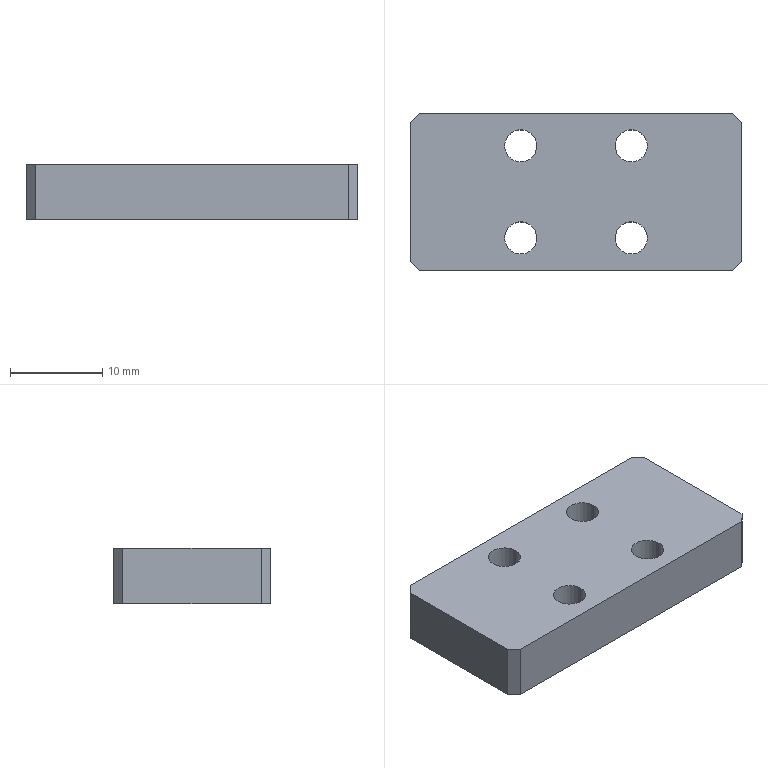Component | SolidWorks | ClampC-1 | 1 solid | 18 faces | box 36 x 17 x 6 mm | volume 3429 mm3 | plane 10 | cylinder 8 | commonest cylinder face diameters 3.5 x8
build123d program:
from build123d import *

# Parameters (mm, degrees)
SKETCH1_W                  = 36
SKETCH1_H                  = 17
EXTRUDE1_DEPTH             = 6
F_3_5_3_5_DIAMETER_HOLE1_D = 3.5
CHAMFER1_SIZE              = 1


with BuildPart() as part:
    # Sketch1 → Extrude1 (new body)
    with BuildSketch(Plane.XY):
        Rectangle(SKETCH1_W, SKETCH1_H)
    extrude(amount=EXTRUDE1_DEPTH)

    # 3.5 _3.5_ Diameter Hole1 (through all)
    with Locations(Plane.XY.offset(6)):
        with Locations((-6, 5), (6, 5), (6, -5), (-6, -5)):
            Hole(F_3_5_3_5_DIAMETER_HOLE1_D / 2)

    # Chamfer1
    chamfer1_edges = [part.edges().sort_by_distance(p)[0] for p in [
        (-18, 8.5, 3),
        (18, 8.5, 3),
        (18, -8.5, 3),
        (-18, -8.5, 3),
    ]]
    chamfer(chamfer1_edges, length=CHAMFER1_SIZE)


solid = part.part

# Placed as in the assembly
solid = solid.moved(Location((13, 29, 10), (0, 0, 0)))
STEP:
#1=CARTESIAN_POINT('',(0.2067,1.339,0.3937));
#2=VERTEX_POINT('',#1);
#3=CARTESIAN_POINT('',(0.3445,1.339,0.3937));
#4=VERTEX_POINT('',#3);
#5=CARTESIAN_POINT('',(0.2756,1.339,0.3937));
#6=DIRECTION('',(0.,0.,1.));
#7=DIRECTION('',(1.,0.,0.));
#8=AXIS2_PLACEMENT_3D('',#5,#6,#7);
#9=CIRCLE('',#8,0.0689);
#10=EDGE_CURVE('',#2,#4,#9,.T.);
#11=ORIENTED_EDGE('',*,*,#10,.F.);
#12=CARTESIAN_POINT('',(0.2067,1.339,0.6299));
#13=VERTEX_POINT('',#12);
#14=CARTESIAN_POINT('',(0.2067,1.339,0.6299));
#15=DIRECTION('',(0.,0.,1.));
#16=VECTOR('',#15,39.37);
#17=LINE('',#14,#16);
#18=EDGE_CURVE('',#2,#13,#17,.T.);
#19=ORIENTED_EDGE('',*,*,#18,.T.);
#20=CARTESIAN_POINT('',(0.3445,1.339,0.6299));
#21=VERTEX_POINT('',#20);
#22=CARTESIAN_POINT('',(0.2756,1.339,0.6299));
#23=DIRECTION('',(0.,0.,1.));
#24=DIRECTION('',(1.,0.,0.));
#25=AXIS2_PLACEMENT_3D('',#22,#23,#24);
#26=CIRCLE('',#25,0.0689);
#27=EDGE_CURVE('',#13,#21,#26,.T.);
#28=ORIENTED_EDGE('',*,*,#27,.T.);
#29=CARTESIAN_POINT('',(0.3445,1.339,0.6299));
#30=DIRECTION('',(0.,0.,1.));
#31=VECTOR('',#30,39.37);
#32=LINE('',#29,#31);
#33=EDGE_CURVE('',#4,#21,#32,.T.);
#34=ORIENTED_EDGE('',*,*,#33,.F.);
#35=EDGE_LOOP('',(#11,#19,#28,#34));
#36=FACE_OUTER_BOUND('',#35,.T.);
#37=CARTESIAN_POINT('',(0.2756,1.339,0.6299));
#38=DIRECTION('',(0.,0.,1.));
#39=DIRECTION('',(1.,0.,0.));
#40=AXIS2_PLACEMENT_3D('',#37,#38,#39);
#41=CYLINDRICAL_SURFACE('',#40,0.0689);
#42=ADVANCED_FACE('',(#36),#41,.F.);
#43=CARTESIAN_POINT('',(0.6791,1.339,0.3937));
#44=VERTEX_POINT('',#43);
#45=CARTESIAN_POINT('',(0.8169,1.339,0.3937));
#46=VERTEX_POINT('',#45);
#47=CARTESIAN_POINT('',(0.748,1.339,0.3937));
#48=DIRECTION('',(0.,0.,1.));
#49=DIRECTION('',(1.,0.,0.));
#50=AXIS2_PLACEMENT_3D('',#47,#48,#49);
#51=CIRCLE('',#50,0.0689);
#52=EDGE_CURVE('',#44,#46,#51,.T.);
#53=ORIENTED_EDGE('',*,*,#52,.F.);
#54=CARTESIAN_POINT('',(0.6791,1.339,0.6299));
#55=VERTEX_POINT('',#54);
#56=CARTESIAN_POINT('',(0.6791,1.339,0.6299));
#57=DIRECTION('',(0.,0.,1.));
#58=VECTOR('',#57,39.37);
#59=LINE('',#56,#58);
#60=EDGE_CURVE('',#44,#55,#59,.T.);
#61=ORIENTED_EDGE('',*,*,#60,.T.);
#62=CARTESIAN_POINT('',(0.8169,1.339,0.6299));
#63=VERTEX_POINT('',#62);
#64=CARTESIAN_POINT('',(0.748,1.339,0.6299));
#65=DIRECTION('',(0.,0.,1.));
#66=DIRECTION('',(1.,0.,0.));
#67=AXIS2_PLACEMENT_3D('',#64,#65,#66);
#68=CIRCLE('',#67,0.0689);
#69=EDGE_CURVE('',#55,#63,#68,.T.);
#70=ORIENTED_EDGE('',*,*,#69,.T.);
#71=CARTESIAN_POINT('',(0.8169,1.339,0.6299));
#72=DIRECTION('',(0.,0.,1.));
#73=VECTOR('',#72,39.37);
#74=LINE('',#71,#73);
#75=EDGE_CURVE('',#46,#63,#74,.T.);
#76=ORIENTED_EDGE('',*,*,#75,.F.);
#77=EDGE_LOOP('',(#53,#61,#70,#76));
#78=FACE_OUTER_BOUND('',#77,.T.);
#79=CARTESIAN_POINT('',(0.748,1.339,0.6299));
#80=DIRECTION('',(0.,0.,1.));
#81=DIRECTION('',(1.,0.,0.));
#82=AXIS2_PLACEMENT_3D('',#79,#80,#81);
#83=CYLINDRICAL_SURFACE('',#82,0.0689);
#84=ADVANCED_FACE('',(#78),#83,.F.);
#85=CARTESIAN_POINT('',(0.6791,0.9449,0.3937));
#86=VERTEX_POINT('',#85);
#87=CARTESIAN_POINT('',(0.8169,0.9449,0.3937));
#88=VERTEX_POINT('',#87);
#89=CARTESIAN_POINT('',(0.748,0.9449,0.3937));
#90=DIRECTION('',(0.,0.,1.));
#91=DIRECTION('',(1.,0.,0.));
#92=AXIS2_PLACEMENT_3D('',#89,#90,#91);
#93=CIRCLE('',#92,0.0689);
#94=EDGE_CURVE('',#86,#88,#93,.T.);
#95=ORIENTED_EDGE('',*,*,#94,.F.);
#96=CARTESIAN_POINT('',(0.6791,0.9449,0.6299));
#97=VERTEX_POINT('',#96);
#98=CARTESIAN_POINT('',(0.6791,0.9449,0.6299));
#99=DIRECTION('',(0.,0.,1.));
#100=VECTOR('',#99,39.37);
#101=LINE('',#98,#100);
#102=EDGE_CURVE('',#86,#97,#101,.T.);
#103=ORIENTED_EDGE('',*,*,#102,.T.);
#104=CARTESIAN_POINT('',(0.8169,0.9449,0.6299));
#105=VERTEX_POINT('',#104);
#106=CARTESIAN_POINT('',(0.748,0.9449,0.6299));
#107=DIRECTION('',(0.,0.,1.));
#108=DIRECTION('',(1.,0.,0.));
#109=AXIS2_PLACEMENT_3D('',#106,#107,#108);
#110=CIRCLE('',#109,0.0689);
#111=EDGE_CURVE('',#97,#105,#110,.T.);
#112=ORIENTED_EDGE('',*,*,#111,.T.);
#113=CARTESIAN_POINT('',(0.8169,0.9449,0.6299));
#114=DIRECTION('',(0.,0.,1.));
#115=VECTOR('',#114,39.37);
#116=LINE('',#113,#115);
#117=EDGE_CURVE('',#88,#105,#116,.T.);
#118=ORIENTED_EDGE('',*,*,#117,.F.);
#119=EDGE_LOOP('',(#95,#103,#112,#118));
#120=FACE_OUTER_BOUND('',#119,.T.);
#121=CARTESIAN_POINT('',(0.748,0.9449,0.6299));
#122=DIRECTION('',(0.,0.,1.));
#123=DIRECTION('',(1.,0.,0.));
#124=AXIS2_PLACEMENT_3D('',#121,#122,#123);
#125=CYLINDRICAL_SURFACE('',#124,0.0689);
#126=ADVANCED_FACE('',(#120),#125,.F.);
#127=CARTESIAN_POINT('',(0.2067,0.9449,0.3937));
#128=VERTEX_POINT('',#127);
#129=CARTESIAN_POINT('',(0.3445,0.9449,0.3937));
#130=VERTEX_POINT('',#129);
#131=CARTESIAN_POINT('',(0.2756,0.9449,0.3937));
#132=DIRECTION('',(0.,0.,1.));
#133=DIRECTION('',(1.,0.,0.));
#134=AXIS2_PLACEMENT_3D('',#131,#132,#133);
#135=CIRCLE('',#134,0.0689);
#136=EDGE_CURVE('',#128,#130,#135,.T.);
#137=ORIENTED_EDGE('',*,*,#136,.F.);
#138=CARTESIAN_POINT('',(0.2067,0.9449,0.6299));
#139=VERTEX_POINT('',#138);
#140=CARTESIAN_POINT('',(0.2067,0.9449,0.6299));
#141=DIRECTION('',(0.,0.,1.));
#142=VECTOR('',#141,39.37);
#143=LINE('',#140,#142);
#144=EDGE_CURVE('',#128,#139,#143,.T.);
#145=ORIENTED_EDGE('',*,*,#144,.T.);
#146=CARTESIAN_POINT('',(0.3445,0.9449,0.6299));
#147=VERTEX_POINT('',#146);
#148=CARTESIAN_POINT('',(0.2756,0.9449,0.6299));
#149=DIRECTION('',(0.,0.,1.));
#150=DIRECTION('',(1.,0.,0.));
#151=AXIS2_PLACEMENT_3D('',#148,#149,#150);
#152=CIRCLE('',#151,0.0689);
#153=EDGE_CURVE('',#139,#147,#152,.T.);
#154=ORIENTED_EDGE('',*,*,#153,.T.);
#155=CARTESIAN_POINT('',(0.3445,0.9449,0.6299));
#156=DIRECTION('',(0.,0.,1.));
#157=VECTOR('',#156,39.37);
#158=LINE('',#155,#157);
#159=EDGE_CURVE('',#130,#147,#158,.T.);
#160=ORIENTED_EDGE('',*,*,#159,.F.);
#161=EDGE_LOOP('',(#137,#145,#154,#160));
#162=FACE_OUTER_BOUND('',#161,.T.);
#163=CARTESIAN_POINT('',(0.2756,0.9449,0.6299));
#164=DIRECTION('',(0.,0.,1.));
#165=DIRECTION('',(1.,0.,0.));
#166=AXIS2_PLACEMENT_3D('',#163,#164,#165);
#167=CYLINDRICAL_SURFACE('',#166,0.0689);
#168=ADVANCED_FACE('',(#162),#167,.F.);
#169=CARTESIAN_POINT('',(-0.1969,1.437,0.3937));
#170=VERTEX_POINT('',#169);
#171=CARTESIAN_POINT('',(-0.1969,0.8465,0.3937));
#172=VERTEX_POINT('',#171);
#173=CARTESIAN_POINT('',(-0.1969,0.8071,0.3937));
#174=DIRECTION('',(0.,-1.,0.));
#175=VECTOR('',#174,39.37);
#176=LINE('',#173,#175);
#177=EDGE_CURVE('',#170,#172,#176,.T.);
#178=ORIENTED_EDGE('',*,*,#177,.T.);
#179=CARTESIAN_POINT('',(-0.1969,0.8465,0.6299));
#180=VERTEX_POINT('',#179);
#181=CARTESIAN_POINT('',(-0.1969,0.8465,0.6299));
#182=DIRECTION('',(0.,0.,1.));
#183=VECTOR('',#182,39.37);
#184=LINE('',#181,#183);
#185=EDGE_CURVE('',#172,#180,#184,.T.);
#186=ORIENTED_EDGE('',*,*,#185,.T.);
#187=CARTESIAN_POINT('',(-0.1969,1.437,0.6299));
#188=VERTEX_POINT('',#187);
#189=CARTESIAN_POINT('',(-0.1969,0.8071,0.6299));
#190=DIRECTION('',(0.,-1.,0.));
#191=VECTOR('',#190,39.37);
#192=LINE('',#189,#191);
#193=EDGE_CURVE('',#188,#180,#192,.T.);
#194=ORIENTED_EDGE('',*,*,#193,.F.);
#195=CARTESIAN_POINT('',(-0.1969,1.437,0.6299));
#196=DIRECTION('',(0.,0.,-1.));
#197=VECTOR('',#196,39.37);
#198=LINE('',#195,#197);
#199=EDGE_CURVE('',#188,#170,#198,.T.);
#200=ORIENTED_EDGE('',*,*,#199,.T.);
#201=EDGE_LOOP('',(#178,#186,#194,#200));
#202=FACE_OUTER_BOUND('',#201,.T.);
#203=CARTESIAN_POINT('',(-0.1969,0.8071,0.6299));
#204=DIRECTION('',(1.,0.,0.));
#205=DIRECTION('',(0.,0.,-1.));
#206=AXIS2_PLACEMENT_3D('',#203,#204,#205);
#207=PLANE('',#206);
#208=ADVANCED_FACE('',(#202),#207,.F.);
#209=CARTESIAN_POINT('',(-0.1575,0.8071,0.3937));
#210=VERTEX_POINT('',#209);
#211=CARTESIAN_POINT('',(1.181,0.8071,0.3937));
#212=VERTEX_POINT('',#211);
#213=CARTESIAN_POINT('',(1.22,0.8071,0.3937));
#214=DIRECTION('',(1.,0.,0.));
#215=VECTOR('',#214,39.37);
#216=LINE('',#213,#215);
#217=EDGE_CURVE('',#210,#212,#216,.T.);
#218=ORIENTED_EDGE('',*,*,#217,.T.);
#219=CARTESIAN_POINT('',(1.181,0.8071,0.6299));
#220=VERTEX_POINT('',#219);
#221=CARTESIAN_POINT('',(1.181,0.8071,0.6299));
#222=DIRECTION('',(0.,0.,1.));
#223=VECTOR('',#222,39.37);
#224=LINE('',#221,#223);
#225=EDGE_CURVE('',#212,#220,#224,.T.);
#226=ORIENTED_EDGE('',*,*,#225,.T.);
#227=CARTESIAN_POINT('',(-0.1575,0.8071,0.6299));
#228=VERTEX_POINT('',#227);
#229=CARTESIAN_POINT('',(1.22,0.8071,0.6299));
#230=DIRECTION('',(1.,0.,0.));
#231=VECTOR('',#230,39.37);
#232=LINE('',#229,#231);
#233=EDGE_CURVE('',#228,#220,#232,.T.);
#234=ORIENTED_EDGE('',*,*,#233,.F.);
#235=CARTESIAN_POINT('',(-0.1575,0.8071,0.6299));
#236=DIRECTION('',(0.,0.,-1.));
#237=VECTOR('',#236,39.37);
#238=LINE('',#235,#237);
#239=EDGE_CURVE('',#228,#210,#238,.T.);
#240=ORIENTED_EDGE('',*,*,#239,.T.);
#241=EDGE_LOOP('',(#218,#226,#234,#240));
#242=FACE_OUTER_BOUND('',#241,.T.);
#243=CARTESIAN_POINT('',(1.22,0.8071,0.6299));
#244=DIRECTION('',(-0.,1.,0.));
#245=DIRECTION('',(-1.,-0.,0.));
#246=AXIS2_PLACEMENT_3D('',#243,#244,#245);
#247=PLANE('',#246);
#248=ADVANCED_FACE('',(#242),#247,.F.);
#249=CARTESIAN_POINT('',(1.22,0.8465,0.6299));
#250=VERTEX_POINT('',#249);
#251=CARTESIAN_POINT('',(1.22,1.437,0.6299));
#252=VERTEX_POINT('',#251);
#253=CARTESIAN_POINT('',(1.22,0.8071,0.6299));
#254=DIRECTION('',(0.,1.,0.));
#255=VECTOR('',#254,39.37);
#256=LINE('',#253,#255);
#257=EDGE_CURVE('',#250,#252,#256,.T.);
#258=ORIENTED_EDGE('',*,*,#257,.F.);
#259=CARTESIAN_POINT('',(1.22,0.8465,0.3937));
#260=VERTEX_POINT('',#259);
#261=CARTESIAN_POINT('',(1.22,0.8465,0.6299));
#262=DIRECTION('',(0.,0.,-1.));
#263=VECTOR('',#262,39.37);
#264=LINE('',#261,#263);
#265=EDGE_CURVE('',#250,#260,#264,.T.);
#266=ORIENTED_EDGE('',*,*,#265,.T.);
#267=CARTESIAN_POINT('',(1.22,1.437,0.3937));
#268=VERTEX_POINT('',#267);
#269=CARTESIAN_POINT('',(1.22,0.8071,0.3937));
#270=DIRECTION('',(0.,1.,0.));
#271=VECTOR('',#270,39.37);
#272=LINE('',#269,#271);
#273=EDGE_CURVE('',#260,#268,#272,.T.);
#274=ORIENTED_EDGE('',*,*,#273,.T.);
#275=CARTESIAN_POINT('',(1.22,1.437,0.6299));
#276=DIRECTION('',(0.,0.,1.));
#277=VECTOR('',#276,39.37);
#278=LINE('',#275,#277);
#279=EDGE_CURVE('',#268,#252,#278,.T.);
#280=ORIENTED_EDGE('',*,*,#279,.T.);
#281=EDGE_LOOP('',(#258,#266,#274,#280));
#282=FACE_OUTER_BOUND('',#281,.T.);
#283=CARTESIAN_POINT('',(1.22,0.8071,0.6299));
#284=DIRECTION('',(-1.,0.,0.));
#285=DIRECTION('',(0.,0.,1.));
#286=AXIS2_PLACEMENT_3D('',#283,#284,#285);
#287=PLANE('',#286);
#288=ADVANCED_FACE('',(#282),#287,.F.);
#289=CARTESIAN_POINT('',(1.181,1.476,0.6299));
#290=VERTEX_POINT('',#289);
#291=CARTESIAN_POINT('',(-0.1575,1.476,0.6299));
#292=VERTEX_POINT('',#291);
#293=CARTESIAN_POINT('',(1.22,1.476,0.6299));
#294=DIRECTION('',(-1.,-0.,0.));
#295=VECTOR('',#294,39.37);
#296=LINE('',#293,#295);
#297=EDGE_CURVE('',#290,#292,#296,.T.);
#298=ORIENTED_EDGE('',*,*,#297,.F.);
#299=CARTESIAN_POINT('',(1.181,1.476,0.3937));
#300=VERTEX_POINT('',#299);
#301=CARTESIAN_POINT('',(1.181,1.476,0.6299));
#302=DIRECTION('',(0.,0.,-1.));
#303=VECTOR('',#302,39.37);
#304=LINE('',#301,#303);
#305=EDGE_CURVE('',#290,#300,#304,.T.);
#306=ORIENTED_EDGE('',*,*,#305,.T.);
#307=CARTESIAN_POINT('',(-0.1575,1.476,0.3937));
#308=VERTEX_POINT('',#307);
#309=CARTESIAN_POINT('',(1.22,1.476,0.3937));
#310=DIRECTION('',(-1.,-0.,0.));
#311=VECTOR('',#310,39.37);
#312=LINE('',#309,#311);
#313=EDGE_CURVE('',#300,#308,#312,.T.);
#314=ORIENTED_EDGE('',*,*,#313,.T.);
#315=CARTESIAN_POINT('',(-0.1575,1.476,0.6299));
#316=DIRECTION('',(0.,0.,1.));
#317=VECTOR('',#316,39.37);
#318=LINE('',#315,#317);
#319=EDGE_CURVE('',#308,#292,#318,.T.);
#320=ORIENTED_EDGE('',*,*,#319,.T.);
#321=EDGE_LOOP('',(#298,#306,#314,#320));
#322=FACE_OUTER_BOUND('',#321,.T.);
#323=CARTESIAN_POINT('',(1.22,1.476,0.6299));
#324=DIRECTION('',(0.,-1.,0.));
#325=DIRECTION('',(1.,0.,0.));
#326=AXIS2_PLACEMENT_3D('',#323,#324,#325);
#327=PLANE('',#326);
#328=ADVANCED_FACE('',(#322),#327,.F.);
#329=CARTESIAN_POINT('',(0.2756,1.339,0.6299));
#330=DIRECTION('',(0.,0.,1.));
#331=DIRECTION('',(1.,0.,0.));
#332=AXIS2_PLACEMENT_3D('',#329,#330,#331);
#333=CIRCLE('',#332,0.0689);
#334=EDGE_CURVE('',#21,#13,#333,.T.);
#335=ORIENTED_EDGE('',*,*,#334,.F.);
#336=ORIENTED_EDGE('',*,*,#27,.F.);
#337=EDGE_LOOP('',(#335,#336));
#338=FACE_BOUND('',#337,.T.);
#339=CARTESIAN_POINT('',(0.748,1.339,0.6299));
#340=DIRECTION('',(0.,0.,1.));
#341=DIRECTION('',(1.,0.,0.));
#342=AXIS2_PLACEMENT_3D('',#339,#340,#341);
#343=CIRCLE('',#342,0.0689);
#344=EDGE_CURVE('',#63,#55,#343,.T.);
#345=ORIENTED_EDGE('',*,*,#344,.F.);
#346=ORIENTED_EDGE('',*,*,#69,.F.);
#347=EDGE_LOOP('',(#345,#346));
#348=FACE_BOUND('',#347,.T.);
#349=CARTESIAN_POINT('',(0.748,0.9449,0.6299));
#350=DIRECTION('',(0.,0.,1.));
#351=DIRECTION('',(1.,0.,0.));
#352=AXIS2_PLACEMENT_3D('',#349,#350,#351);
#353=CIRCLE('',#352,0.0689);
#354=EDGE_CURVE('',#105,#97,#353,.T.);
#355=ORIENTED_EDGE('',*,*,#354,.F.);
#356=ORIENTED_EDGE('',*,*,#111,.F.);
#357=EDGE_LOOP('',(#355,#356));
#358=FACE_BOUND('',#357,.T.);
#359=CARTESIAN_POINT('',(0.2756,0.9449,0.6299));
#360=DIRECTION('',(0.,0.,1.));
#361=DIRECTION('',(1.,0.,0.));
#362=AXIS2_PLACEMENT_3D('',#359,#360,#361);
#363=CIRCLE('',#362,0.0689);
#364=EDGE_CURVE('',#147,#139,#363,.T.);
#365=ORIENTED_EDGE('',*,*,#364,.F.);
#366=ORIENTED_EDGE('',*,*,#153,.F.);
#367=EDGE_LOOP('',(#365,#366));
#368=FACE_BOUND('',#367,.T.);
#369=ORIENTED_EDGE('',*,*,#233,.T.);
#370=CARTESIAN_POINT('',(0.8268,0.4528,0.6299));
#371=DIRECTION('',(0.7071,0.7071,0.));
#372=VECTOR('',#371,39.37);
#373=LINE('',#370,#372);
#374=EDGE_CURVE('',#220,#250,#373,.T.);
#375=ORIENTED_EDGE('',*,*,#374,.T.);
#376=ORIENTED_EDGE('',*,*,#257,.T.);
#377=CARTESIAN_POINT('',(0.4921,2.165,0.6299));
#378=DIRECTION('',(-0.7071,0.7071,0.));
#379=VECTOR('',#378,39.37);
#380=LINE('',#377,#379);
#381=EDGE_CURVE('',#252,#290,#380,.T.);
#382=ORIENTED_EDGE('',*,*,#381,.T.);
#383=ORIENTED_EDGE('',*,*,#297,.T.);
#384=CARTESIAN_POINT('',(-0.1772,1.457,0.6299));
#385=DIRECTION('',(-0.7071,-0.7071,0.));
#386=VECTOR('',#385,39.37);
#387=LINE('',#384,#386);
#388=EDGE_CURVE('',#292,#188,#387,.T.);
#389=ORIENTED_EDGE('',*,*,#388,.T.);
#390=ORIENTED_EDGE('',*,*,#193,.T.);
#391=CARTESIAN_POINT('',(-0.5118,1.161,0.6299));
#392=DIRECTION('',(0.7071,-0.7071,0.));
#393=VECTOR('',#392,39.37);
#394=LINE('',#391,#393);
#395=EDGE_CURVE('',#180,#228,#394,.T.);
#396=ORIENTED_EDGE('',*,*,#395,.T.);
#397=EDGE_LOOP('',(#369,#375,#376,#382,#383,#389,#390,#396));
#398=FACE_OUTER_BOUND('',#397,.T.);
#399=CARTESIAN_POINT('',(-0.1969,1.476,0.6299));
#400=DIRECTION('',(0.,0.,1.));
#401=DIRECTION('',(1.,0.,0.));
#402=AXIS2_PLACEMENT_3D('',#399,#400,#401);
#403=PLANE('',#402);
#404=ADVANCED_FACE('',(#338,#348,#358,#368,#398),#403,.T.);
#405=CARTESIAN_POINT('',(0.2756,1.339,0.3937));
#406=DIRECTION('',(0.,0.,1.));
#407=DIRECTION('',(1.,0.,0.));
#408=AXIS2_PLACEMENT_3D('',#405,#406,#407);
#409=CIRCLE('',#408,0.0689);
#410=EDGE_CURVE('',#4,#2,#409,.T.);
#411=ORIENTED_EDGE('',*,*,#410,.T.);
#412=ORIENTED_EDGE('',*,*,#10,.T.);
#413=EDGE_LOOP('',(#411,#412));
#414=FACE_BOUND('',#413,.T.);
#415=CARTESIAN_POINT('',(0.748,1.339,0.3937));
#416=DIRECTION('',(0.,0.,1.));
#417=DIRECTION('',(1.,0.,0.));
#418=AXIS2_PLACEMENT_3D('',#415,#416,#417);
#419=CIRCLE('',#418,0.0689);
#420=EDGE_CURVE('',#46,#44,#419,.T.);
#421=ORIENTED_EDGE('',*,*,#420,.T.);
#422=ORIENTED_EDGE('',*,*,#52,.T.);
#423=EDGE_LOOP('',(#421,#422));
#424=FACE_BOUND('',#423,.T.);
#425=CARTESIAN_POINT('',(0.748,0.9449,0.3937));
#426=DIRECTION('',(0.,0.,1.));
#427=DIRECTION('',(1.,0.,0.));
#428=AXIS2_PLACEMENT_3D('',#425,#426,#427);
#429=CIRCLE('',#428,0.0689);
#430=EDGE_CURVE('',#88,#86,#429,.T.);
#431=ORIENTED_EDGE('',*,*,#430,.T.);
#432=ORIENTED_EDGE('',*,*,#94,.T.);
#433=EDGE_LOOP('',(#431,#432));
#434=FACE_BOUND('',#433,.T.);
#435=CARTESIAN_POINT('',(0.2756,0.9449,0.3937));
#436=DIRECTION('',(0.,0.,1.));
#437=DIRECTION('',(1.,0.,0.));
#438=AXIS2_PLACEMENT_3D('',#435,#436,#437);
#439=CIRCLE('',#438,0.0689);
#440=EDGE_CURVE('',#130,#128,#439,.T.);
#441=ORIENTED_EDGE('',*,*,#440,.T.);
#442=ORIENTED_EDGE('',*,*,#136,.T.);
#443=EDGE_LOOP('',(#441,#442));
#444=FACE_BOUND('',#443,.T.);
#445=ORIENTED_EDGE('',*,*,#273,.F.);
#446=CARTESIAN_POINT('',(1.22,0.8465,0.3937));
#447=DIRECTION('',(-0.7071,-0.7071,0.));
#448=VECTOR('',#447,39.37);
#449=LINE('',#446,#448);
#450=EDGE_CURVE('',#260,#212,#449,.T.);
#451=ORIENTED_EDGE('',*,*,#450,.T.);
#452=ORIENTED_EDGE('',*,*,#217,.F.);
#453=CARTESIAN_POINT('',(-0.1575,0.8071,0.3937));
#454=DIRECTION('',(-0.7071,0.7071,0.));
#455=VECTOR('',#454,39.37);
#456=LINE('',#453,#455);
#457=EDGE_CURVE('',#210,#172,#456,.T.);
#458=ORIENTED_EDGE('',*,*,#457,.T.);
#459=ORIENTED_EDGE('',*,*,#177,.F.);
#460=CARTESIAN_POINT('',(-0.1969,1.437,0.3937));
#461=DIRECTION('',(0.7071,0.7071,0.));
#462=VECTOR('',#461,39.37);
#463=LINE('',#460,#462);
#464=EDGE_CURVE('',#170,#308,#463,.T.);
#465=ORIENTED_EDGE('',*,*,#464,.T.);
#466=ORIENTED_EDGE('',*,*,#313,.F.);
#467=CARTESIAN_POINT('',(1.181,1.476,0.3937));
#468=DIRECTION('',(0.7071,-0.7071,0.));
#469=VECTOR('',#468,39.37);
#470=LINE('',#467,#469);
#471=EDGE_CURVE('',#300,#268,#470,.T.);
#472=ORIENTED_EDGE('',*,*,#471,.T.);
#473=EDGE_LOOP('',(#445,#451,#452,#458,#459,#465,#466,#472));
#474=FACE_OUTER_BOUND('',#473,.T.);
#475=CARTESIAN_POINT('',(-0.1969,1.476,0.3937));
#476=DIRECTION('',(0.,0.,1.));
#477=DIRECTION('',(1.,0.,0.));
#478=AXIS2_PLACEMENT_3D('',#475,#476,#477);
#479=PLANE('',#478);
#480=ADVANCED_FACE('',(#414,#424,#434,#444,#474),#479,.F.);
#481=ORIENTED_EDGE('',*,*,#144,.F.);
#482=ORIENTED_EDGE('',*,*,#440,.F.);
#483=ORIENTED_EDGE('',*,*,#159,.T.);
#484=ORIENTED_EDGE('',*,*,#364,.T.);
#485=EDGE_LOOP('',(#481,#482,#483,#484));
#486=FACE_OUTER_BOUND('',#485,.T.);
#487=CARTESIAN_POINT('',(0.2756,0.9449,0.6299));
#488=DIRECTION('',(0.,0.,1.));
#489=DIRECTION('',(1.,0.,0.));
#490=AXIS2_PLACEMENT_3D('',#487,#488,#489);
#491=CYLINDRICAL_SURFACE('',#490,0.0689);
#492=ADVANCED_FACE('',(#486),#491,.F.);
#493=ORIENTED_EDGE('',*,*,#102,.F.);
#494=ORIENTED_EDGE('',*,*,#430,.F.);
#495=ORIENTED_EDGE('',*,*,#117,.T.);
#496=ORIENTED_EDGE('',*,*,#354,.T.);
#497=EDGE_LOOP('',(#493,#494,#495,#496));
#498=FACE_OUTER_BOUND('',#497,.T.);
#499=CARTESIAN_POINT('',(0.748,0.9449,0.6299));
#500=DIRECTION('',(0.,0.,1.));
#501=DIRECTION('',(1.,0.,0.));
#502=AXIS2_PLACEMENT_3D('',#499,#500,#501);
#503=CYLINDRICAL_SURFACE('',#502,0.0689);
#504=ADVANCED_FACE('',(#498),#503,.F.);
#505=ORIENTED_EDGE('',*,*,#60,.F.);
#506=ORIENTED_EDGE('',*,*,#420,.F.);
#507=ORIENTED_EDGE('',*,*,#75,.T.);
#508=ORIENTED_EDGE('',*,*,#344,.T.);
#509=EDGE_LOOP('',(#505,#506,#507,#508));
#510=FACE_OUTER_BOUND('',#509,.T.);
#511=CARTESIAN_POINT('',(0.748,1.339,0.6299));
#512=DIRECTION('',(0.,0.,1.));
#513=DIRECTION('',(1.,0.,0.));
#514=AXIS2_PLACEMENT_3D('',#511,#512,#513);
#515=CYLINDRICAL_SURFACE('',#514,0.0689);
#516=ADVANCED_FACE('',(#510),#515,.F.);
#517=ORIENTED_EDGE('',*,*,#18,.F.);
#518=ORIENTED_EDGE('',*,*,#410,.F.);
#519=ORIENTED_EDGE('',*,*,#33,.T.);
#520=ORIENTED_EDGE('',*,*,#334,.T.);
#521=EDGE_LOOP('',(#517,#518,#519,#520));
#522=FACE_OUTER_BOUND('',#521,.T.);
#523=CARTESIAN_POINT('',(0.2756,1.339,0.6299));
#524=DIRECTION('',(0.,0.,1.));
#525=DIRECTION('',(1.,0.,0.));
#526=AXIS2_PLACEMENT_3D('',#523,#524,#525);
#527=CYLINDRICAL_SURFACE('',#526,0.0689);
#528=ADVANCED_FACE('',(#522),#527,.F.);
#529=ORIENTED_EDGE('',*,*,#374,.F.);
#530=ORIENTED_EDGE('',*,*,#225,.F.);
#531=ORIENTED_EDGE('',*,*,#450,.F.);
#532=ORIENTED_EDGE('',*,*,#265,.F.);
#533=EDGE_LOOP('',(#529,#530,#531,#532));
#534=FACE_OUTER_BOUND('',#533,.T.);
#535=CARTESIAN_POINT('',(1.22,0.8465,0.6299));
#536=DIRECTION('',(-0.7071,0.7071,0.));
#537=DIRECTION('',(-0.7071,-0.7071,0.));
#538=AXIS2_PLACEMENT_3D('',#535,#536,#537);
#539=PLANE('',#538);
#540=ADVANCED_FACE('',(#534),#539,.F.);
#541=ORIENTED_EDGE('',*,*,#395,.F.);
#542=ORIENTED_EDGE('',*,*,#185,.F.);
#543=ORIENTED_EDGE('',*,*,#457,.F.);
#544=ORIENTED_EDGE('',*,*,#239,.F.);
#545=EDGE_LOOP('',(#541,#542,#543,#544));
#546=FACE_OUTER_BOUND('',#545,.T.);
#547=CARTESIAN_POINT('',(-0.1575,0.8071,0.6299));
#548=DIRECTION('',(0.7071,0.7071,0.));
#549=DIRECTION('',(-0.7071,0.7071,0.));
#550=AXIS2_PLACEMENT_3D('',#547,#548,#549);
#551=PLANE('',#550);
#552=ADVANCED_FACE('',(#546),#551,.F.);
#553=ORIENTED_EDGE('',*,*,#381,.F.);
#554=ORIENTED_EDGE('',*,*,#279,.F.);
#555=ORIENTED_EDGE('',*,*,#471,.F.);
#556=ORIENTED_EDGE('',*,*,#305,.F.);
#557=EDGE_LOOP('',(#553,#554,#555,#556));
#558=FACE_OUTER_BOUND('',#557,.T.);
#559=CARTESIAN_POINT('',(1.181,1.476,0.6299));
#560=DIRECTION('',(-0.7071,-0.7071,0.));
#561=DIRECTION('',(0.7071,-0.7071,0.));
#562=AXIS2_PLACEMENT_3D('',#559,#560,#561);
#563=PLANE('',#562);
#564=ADVANCED_FACE('',(#558),#563,.F.);
#565=ORIENTED_EDGE('',*,*,#388,.F.);
#566=ORIENTED_EDGE('',*,*,#319,.F.);
#567=ORIENTED_EDGE('',*,*,#464,.F.);
#568=ORIENTED_EDGE('',*,*,#199,.F.);
#569=EDGE_LOOP('',(#565,#566,#567,#568));
#570=FACE_OUTER_BOUND('',#569,.T.);
#571=CARTESIAN_POINT('',(-0.1969,1.437,0.6299));
#572=DIRECTION('',(0.7071,-0.7071,0.));
#573=DIRECTION('',(0.7071,0.7071,0.));
#574=AXIS2_PLACEMENT_3D('',#571,#572,#573);
#575=PLANE('',#574);
#576=ADVANCED_FACE('',(#570),#575,.F.);
#577=CLOSED_SHELL('',(#42,#84,#126,#168,#208,#248,#288,#328,#404,#480,#492,#504,#516,#528,#540,#552,#564,#576));
#578=MANIFOLD_SOLID_BREP('',#577);
#579=CARTESIAN_POINT('',(0.,0.,0.));
#580=DIRECTION('',(0.,0.,1.));
#581=DIRECTION('',(1.,0.,0.));
#582=AXIS2_PLACEMENT_3D('',#579,#580,#581);
#583=(LENGTH_UNIT()NAMED_UNIT(*)SI_UNIT($,.METRE.));
#584=LENGTH_MEASURE_WITH_UNIT(LENGTH_MEASURE(0.0254),#583);
#585=DIMENSIONAL_EXPONENTS(1.,0.,0.,0.,0.,0.,0.);
#586=(CONVERSION_BASED_UNIT('',#584)LENGTH_UNIT()NAMED_UNIT(#585));
#587=UNCERTAINTY_MEASURE_WITH_UNIT(LENGTH_MEASURE(0.00001),#586,'','');
#588=(NAMED_UNIT(*)PLANE_ANGLE_UNIT()SI_UNIT($,.RADIAN.));
#589=(NAMED_UNIT(*)SI_UNIT($,.STERADIAN.)SOLID_ANGLE_UNIT());
#590=(GEOMETRIC_REPRESENTATION_CONTEXT(3)GLOBAL_UNCERTAINTY_ASSIGNED_CONTEXT((#587))GLOBAL_UNIT_ASSIGNED_CONTEXT((#586,#588,#589))REPRESENTATION_CONTEXT('',''));
#591=ADVANCED_BREP_SHAPE_REPRESENTATION('',(#578,#582),#590);
#592=COLOUR_RGB('',0.7922,0.8196,0.9333);
#593=FILL_AREA_STYLE_COLOUR('',#592);
#594=FILL_AREA_STYLE('',(#593));
#595=SURFACE_STYLE_FILL_AREA(#594);
#596=SURFACE_SIDE_STYLE('',(#595));
#597=SURFACE_STYLE_USAGE(.BOTH.,#596);
#598=PRESENTATION_STYLE_ASSIGNMENT((#597));
#599=STYLED_ITEM('',(#598),#578);
#600=PRESENTATION_LAYER_ASSIGNMENT('','',(#599));
#601=(LENGTH_UNIT()NAMED_UNIT(*)SI_UNIT($,.METRE.));
#602=LENGTH_MEASURE_WITH_UNIT(LENGTH_MEASURE(0.0254),#601);
#603=DIMENSIONAL_EXPONENTS(1.,0.,0.,0.,0.,0.,0.);
#604=(CONVERSION_BASED_UNIT('',#602)LENGTH_UNIT()NAMED_UNIT(#603));
#605=UNCERTAINTY_MEASURE_WITH_UNIT(LENGTH_MEASURE(0.00001),#604,'','');
#606=(NAMED_UNIT(*)PLANE_ANGLE_UNIT()SI_UNIT($,.RADIAN.));
#607=(NAMED_UNIT(*)SI_UNIT($,.STERADIAN.)SOLID_ANGLE_UNIT());
#608=(GEOMETRIC_REPRESENTATION_CONTEXT(3)GLOBAL_UNCERTAINTY_ASSIGNED_CONTEXT((#605))GLOBAL_UNIT_ASSIGNED_CONTEXT((#604,#606,#607))REPRESENTATION_CONTEXT('',''));
#609=MECHANICAL_DESIGN_GEOMETRIC_PRESENTATION_REPRESENTATION('',(#599),#608);